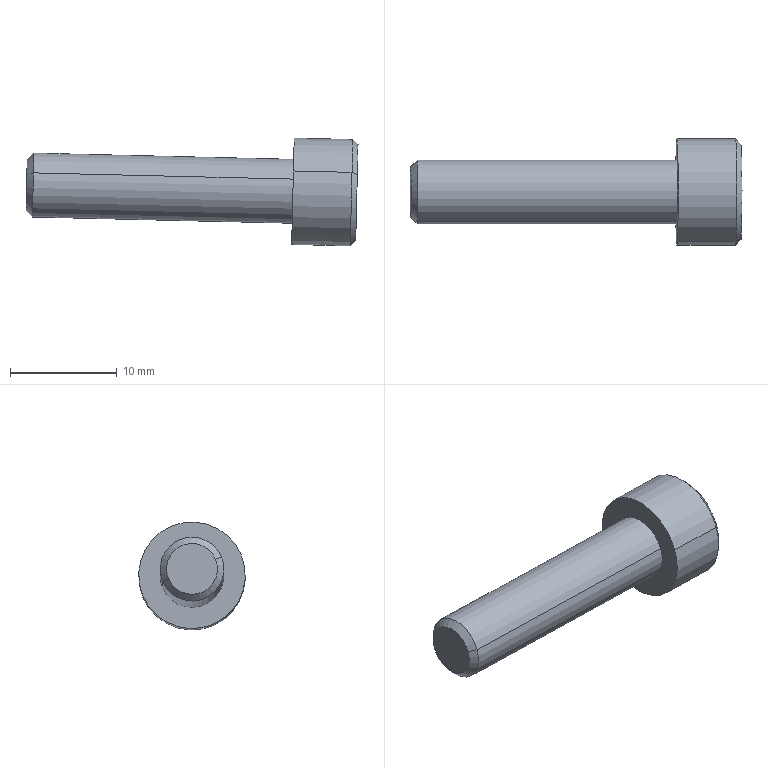Component | SolidWorks | 2012MB0201-1_AUpperRackFrameModule-1_ADJ42-G408-D6.5Assembly-10_HexSocketHeadCapScrewM6-25FerricOxide-1 | 1 solid | 25 faces | box 31.16 x 10 x 10.13 mm | volume 1097 mm3 | plane 15 | cone 6 | cylinder 4 | commonest cylinder face diameters 6 x2 10 x2 | material SCM435
STEP:
#1=COLOUR_RGB('',0.7922,0.8196,0.9333);
#2=FILL_AREA_STYLE_COLOUR('',#1);
#3=FILL_AREA_STYLE('',(#2));
#4=SURFACE_STYLE_FILL_AREA(#3);
#5=SURFACE_SIDE_STYLE('',(#4));
#6=SURFACE_STYLE_USAGE(.BOTH.,#5);
#7=PRESENTATION_STYLE_ASSIGNMENT((#6));
#8=CARTESIAN_POINT('',(-69.831,40.79,-44.912));
#9=VERTEX_POINT('',#8);
#10=CARTESIAN_POINT('',(-69.829,40.616,-44.84));
#11=VERTEX_POINT('',#10);
#12=CARTESIAN_POINT('',(-69.83,40.703,-44.876));
#13=DIRECTION('',(-0.9997,-0.,0.02392));
#14=DIRECTION('',(0.009134,-0.9242,0.3817));
#15=AXIS2_PLACEMENT_3D('',#12,#13,#14);
#16=CIRCLE('',#15,0.0939);
#17=EDGE_CURVE('',#9,#11,#16,.T.);
#18=ORIENTED_EDGE('',*,*,#17,.F.);
#19=CARTESIAN_POINT('',(-69.807,40.812,-44.922));
#20=VERTEX_POINT('',#19);
#21=CARTESIAN_POINT('',(-69.831,40.79,-44.912));
#22=DIRECTION('',(0.7004,0.6535,-0.2868));
#23=VECTOR('',#22,39.37);
#24=LINE('',#21,#23);
#25=EDGE_CURVE('',#9,#20,#24,.T.);
#26=ORIENTED_EDGE('',*,*,#25,.T.);
#27=CARTESIAN_POINT('',(-69.805,40.594,-44.832));
#28=VERTEX_POINT('',#27);
#29=CARTESIAN_POINT('',(-69.806,40.703,-44.877));
#30=DIRECTION('',(0.9997,0.,-0.02392));
#31=DIRECTION('',(0.009134,-0.9242,0.3817));
#32=AXIS2_PLACEMENT_3D('',#29,#30,#31);
#33=CIRCLE('',#32,0.1181);
#34=EDGE_CURVE('',#28,#20,#33,.T.);
#35=ORIENTED_EDGE('',*,*,#34,.F.);
#36=CARTESIAN_POINT('',(-69.829,40.616,-44.84));
#37=DIRECTION('',(0.7134,-0.6535,0.253));
#38=VECTOR('',#37,39.37);
#39=LINE('',#36,#38);
#40=EDGE_CURVE('',#11,#28,#39,.T.);
#41=ORIENTED_EDGE('',*,*,#40,.F.);
#42=EDGE_LOOP('',(#18,#26,#35,#41));
#43=FACE_OUTER_BOUND('',#42,.T.);
#44=CARTESIAN_POINT('',(-69.83,40.703,-44.876));
#45=DIRECTION('',(0.9997,0.,-0.02392));
#46=DIRECTION('',(0.009134,-0.9242,0.3817));
#47=AXIS2_PLACEMENT_3D('',#44,#45,#46);
#48=CONICAL_SURFACE('',#47,0.0939,0.7854);
#49=ADVANCED_FACE('',(#43),#48,.T.);
#50=ORIENTED_EDGE('',*,*,#34,.T.);
#51=CARTESIAN_POINT('',(-68.847,40.812,-44.945));
#52=VERTEX_POINT('',#51);
#53=CARTESIAN_POINT('',(-72.783,40.812,-44.851));
#54=DIRECTION('',(0.9997,0.,-0.02392));
#55=VECTOR('',#54,39.37);
#56=LINE('',#53,#55);
#57=EDGE_CURVE('',#20,#52,#56,.T.);
#58=ORIENTED_EDGE('',*,*,#57,.T.);
#59=CARTESIAN_POINT('',(-68.845,40.594,-44.855));
#60=VERTEX_POINT('',#59);
#61=CARTESIAN_POINT('',(-68.846,40.703,-44.9));
#62=DIRECTION('',(-0.9997,-0.,0.02392));
#63=DIRECTION('',(0.009134,-0.9242,0.3817));
#64=AXIS2_PLACEMENT_3D('',#61,#62,#63);
#65=CIRCLE('',#64,0.1181);
#66=EDGE_CURVE('',#52,#60,#65,.T.);
#67=ORIENTED_EDGE('',*,*,#66,.T.);
#68=CARTESIAN_POINT('',(-72.781,40.594,-44.76));
#69=DIRECTION('',(0.9997,0.,-0.02392));
#70=VECTOR('',#69,39.37);
#71=LINE('',#68,#70);
#72=EDGE_CURVE('',#28,#60,#71,.T.);
#73=ORIENTED_EDGE('',*,*,#72,.F.);
#74=EDGE_LOOP('',(#50,#58,#67,#73));
#75=FACE_OUTER_BOUND('',#74,.T.);
#76=CARTESIAN_POINT('',(-72.782,40.703,-44.806));
#77=DIRECTION('',(0.9997,0.,-0.02392));
#78=DIRECTION('',(0.009134,-0.9242,0.3817));
#79=AXIS2_PLACEMENT_3D('',#76,#77,#78);
#80=CYLINDRICAL_SURFACE('',#79,0.1181);
#81=ADVANCED_FACE('',(#75),#80,.T.);
#82=CARTESIAN_POINT('',(-68.844,40.521,-44.825));
#83=VERTEX_POINT('',#82);
#84=CARTESIAN_POINT('',(-68.848,40.885,-44.975));
#85=VERTEX_POINT('',#84);
#86=CARTESIAN_POINT('',(-68.846,40.703,-44.9));
#87=DIRECTION('',(0.9997,0.,-0.02392));
#88=DIRECTION('',(0.009134,-0.9242,0.3817));
#89=AXIS2_PLACEMENT_3D('',#86,#87,#88);
#90=CIRCLE('',#89,0.1969);
#91=EDGE_CURVE('',#83,#85,#90,.T.);
#92=ORIENTED_EDGE('',*,*,#91,.T.);
#93=CARTESIAN_POINT('',(-68.631,40.885,-44.98));
#94=VERTEX_POINT('',#93);
#95=CARTESIAN_POINT('',(-68.848,40.885,-44.975));
#96=DIRECTION('',(0.9997,0.,-0.02392));
#97=VECTOR('',#96,39.37);
#98=LINE('',#95,#97);
#99=EDGE_CURVE('',#85,#94,#98,.T.);
#100=ORIENTED_EDGE('',*,*,#99,.T.);
#101=CARTESIAN_POINT('',(-68.628,40.521,-44.83));
#102=VERTEX_POINT('',#101);
#103=CARTESIAN_POINT('',(-68.629,40.703,-44.905));
#104=DIRECTION('',(-0.9997,-0.,0.02392));
#105=DIRECTION('',(0.009134,-0.9242,0.3817));
#106=AXIS2_PLACEMENT_3D('',#103,#104,#105);
#107=CIRCLE('',#106,0.1969);
#108=EDGE_CURVE('',#94,#102,#107,.T.);
#109=ORIENTED_EDGE('',*,*,#108,.T.);
#110=CARTESIAN_POINT('',(-68.844,40.521,-44.825));
#111=DIRECTION('',(0.9997,0.,-0.02392));
#112=VECTOR('',#111,39.37);
#113=LINE('',#110,#112);
#114=EDGE_CURVE('',#83,#102,#113,.T.);
#115=ORIENTED_EDGE('',*,*,#114,.F.);
#116=EDGE_LOOP('',(#92,#100,#109,#115));
#117=FACE_OUTER_BOUND('',#116,.T.);
#118=CARTESIAN_POINT('',(-68.846,40.703,-44.9));
#119=DIRECTION('',(0.9997,0.,-0.02392));
#120=DIRECTION('',(0.009134,-0.9242,0.3817));
#121=AXIS2_PLACEMENT_3D('',#118,#119,#120);
#122=CYLINDRICAL_SURFACE('',#121,0.1969);
#123=ADVANCED_FACE('',(#117),#122,.T.);
#124=CARTESIAN_POINT('',(-68.611,40.867,-44.973));
#125=VERTEX_POINT('',#124);
#126=CARTESIAN_POINT('',(-68.608,40.539,-44.838));
#127=VERTEX_POINT('',#126);
#128=CARTESIAN_POINT('',(-68.61,40.703,-44.905));
#129=DIRECTION('',(-0.9997,-0.,0.02392));
#130=DIRECTION('',(-0.009134,0.9242,-0.3817));
#131=AXIS2_PLACEMENT_3D('',#128,#129,#130);
#132=CIRCLE('',#131,0.1772);
#133=EDGE_CURVE('',#125,#127,#132,.T.);
#134=ORIENTED_EDGE('',*,*,#133,.T.);
#135=CARTESIAN_POINT('',(-68.628,40.521,-44.83));
#136=DIRECTION('',(-0.7004,-0.6535,0.2868));
#137=VECTOR('',#136,39.37);
#138=LINE('',#135,#137);
#139=EDGE_CURVE('',#127,#102,#138,.T.);
#140=ORIENTED_EDGE('',*,*,#139,.T.);
#141=ORIENTED_EDGE('',*,*,#108,.F.);
#142=CARTESIAN_POINT('',(-68.631,40.885,-44.98));
#143=DIRECTION('',(-0.7134,0.6535,-0.253));
#144=VECTOR('',#143,39.37);
#145=LINE('',#142,#144);
#146=EDGE_CURVE('',#125,#94,#145,.T.);
#147=ORIENTED_EDGE('',*,*,#146,.F.);
#148=EDGE_LOOP('',(#134,#140,#141,#147));
#149=FACE_OUTER_BOUND('',#148,.T.);
#150=CARTESIAN_POINT('',(-68.629,40.703,-44.905));
#151=DIRECTION('',(-0.9997,-0.,0.02392));
#152=DIRECTION('',(-0.009134,0.9242,-0.3817));
#153=AXIS2_PLACEMENT_3D('',#150,#151,#152);
#154=CONICAL_SURFACE('',#153,0.1969,0.7854);
#155=ADVANCED_FACE('',(#149),#154,.T.);
#156=CARTESIAN_POINT('',(-68.785,40.703,-44.901));
#157=VERTEX_POINT('',#156);
#158=CARTESIAN_POINT('',(-68.727,40.612,-44.865));
#159=VERTEX_POINT('',#158);
#160=CARTESIAN_POINT('',(-68.727,40.612,-44.865));
#161=DIRECTION('',(0.5078,-0.8004,0.3186));
#162=VECTOR('',#161,39.37);
#163=LINE('',#160,#162);
#164=EDGE_CURVE('',#157,#159,#163,.T.);
#165=ORIENTED_EDGE('',*,*,#164,.F.);
#166=CARTESIAN_POINT('',(-68.729,40.794,-44.94));
#167=VERTEX_POINT('',#166);
#168=CARTESIAN_POINT('',(-68.729,40.794,-44.94));
#169=DIRECTION('',(0.4919,0.8004,-0.3426));
#170=VECTOR('',#169,39.37);
#171=LINE('',#168,#170);
#172=EDGE_CURVE('',#157,#167,#171,.T.);
#173=ORIENTED_EDGE('',*,*,#172,.T.);
#174=CARTESIAN_POINT('',(-68.726,40.781,-44.843));
#175=VERTEX_POINT('',#174);
#176=CARTESIAN_POINT('',(-68.728,40.703,-44.903));
#177=DIRECTION('',(-0.9997,-0.,0.02392));
#178=DIRECTION('',(0.009134,-0.9242,0.3817));
#179=AXIS2_PLACEMENT_3D('',#176,#177,#178);
#180=CIRCLE('',#179,0.09843);
#181=EDGE_CURVE('',#175,#167,#180,.T.);
#182=ORIENTED_EDGE('',*,*,#181,.F.);
#183=CARTESIAN_POINT('',(-68.725,40.69,-44.805));
#184=VERTEX_POINT('',#183);
#185=CARTESIAN_POINT('',(-68.728,40.703,-44.903));
#186=DIRECTION('',(-0.9997,-0.,0.02392));
#187=DIRECTION('',(0.009134,-0.9242,0.3817));
#188=AXIS2_PLACEMENT_3D('',#185,#186,#187);
#189=CIRCLE('',#188,0.09843);
#190=EDGE_CURVE('',#184,#175,#189,.T.);
#191=ORIENTED_EDGE('',*,*,#190,.F.);
#192=CARTESIAN_POINT('',(-68.728,40.703,-44.903));
#193=DIRECTION('',(-0.9997,-0.,0.02392));
#194=DIRECTION('',(0.009134,-0.9242,0.3817));
#195=AXIS2_PLACEMENT_3D('',#192,#193,#194);
#196=CIRCLE('',#195,0.09843);
#197=EDGE_CURVE('',#159,#184,#196,.T.);
#198=ORIENTED_EDGE('',*,*,#197,.F.);
#199=EDGE_LOOP('',(#165,#173,#182,#191,#198));
#200=FACE_OUTER_BOUND('',#199,.T.);
#201=CARTESIAN_POINT('',(-68.728,40.703,-44.903));
#202=DIRECTION('',(0.9997,0.,-0.02392));
#203=DIRECTION('',(0.009134,-0.9242,0.3817));
#204=AXIS2_PLACEMENT_3D('',#201,#202,#203);
#205=CONICAL_SURFACE('',#204,0.09843,1.047);
#206=ADVANCED_FACE('',(#200),#205,.F.);
#207=ORIENTED_EDGE('',*,*,#57,.F.);
#208=CARTESIAN_POINT('',(-69.806,40.703,-44.877));
#209=DIRECTION('',(0.9997,0.,-0.02392));
#210=DIRECTION('',(0.009134,-0.9242,0.3817));
#211=AXIS2_PLACEMENT_3D('',#208,#209,#210);
#212=CIRCLE('',#211,0.1181);
#213=EDGE_CURVE('',#20,#28,#212,.T.);
#214=ORIENTED_EDGE('',*,*,#213,.T.);
#215=ORIENTED_EDGE('',*,*,#72,.T.);
#216=CARTESIAN_POINT('',(-68.846,40.703,-44.9));
#217=DIRECTION('',(-0.9997,-0.,0.02392));
#218=DIRECTION('',(0.009134,-0.9242,0.3817));
#219=AXIS2_PLACEMENT_3D('',#216,#217,#218);
#220=CIRCLE('',#219,0.1181);
#221=EDGE_CURVE('',#60,#52,#220,.T.);
#222=ORIENTED_EDGE('',*,*,#221,.T.);
#223=EDGE_LOOP('',(#207,#214,#215,#222));
#224=FACE_OUTER_BOUND('',#223,.T.);
#225=CARTESIAN_POINT('',(-72.782,40.703,-44.806));
#226=DIRECTION('',(0.9997,0.,-0.02392));
#227=DIRECTION('',(0.009134,-0.9242,0.3817));
#228=AXIS2_PLACEMENT_3D('',#225,#226,#227);
#229=CYLINDRICAL_SURFACE('',#228,0.1181);
#230=ADVANCED_FACE('',(#224),#229,.T.);
#231=ORIENTED_EDGE('',*,*,#91,.F.);
#232=CARTESIAN_POINT('',(-68.846,40.703,-44.9));
#233=DIRECTION('',(0.9997,0.,-0.02392));
#234=DIRECTION('',(0.009134,-0.9242,0.3817));
#235=AXIS2_PLACEMENT_3D('',#232,#233,#234);
#236=CIRCLE('',#235,0.1969);
#237=EDGE_CURVE('',#85,#83,#236,.T.);
#238=ORIENTED_EDGE('',*,*,#237,.F.);
#239=EDGE_LOOP('',(#231,#238));
#240=FACE_OUTER_BOUND('',#239,.T.);
#241=ORIENTED_EDGE('',*,*,#221,.F.);
#242=ORIENTED_EDGE('',*,*,#66,.F.);
#243=EDGE_LOOP('',(#241,#242));
#244=FACE_BOUND('',#243,.T.);
#245=CARTESIAN_POINT('',(-68.85,40.628,-45.082));
#246=DIRECTION('',(0.9997,0.,-0.02392));
#247=DIRECTION('',(0.009134,-0.9242,0.3817));
#248=AXIS2_PLACEMENT_3D('',#245,#246,#247);
#249=PLANE('',#248);
#250=ADVANCED_FACE('',(#240,#244),#249,.F.);
#251=ORIENTED_EDGE('',*,*,#99,.F.);
#252=ORIENTED_EDGE('',*,*,#237,.T.);
#253=ORIENTED_EDGE('',*,*,#114,.T.);
#254=CARTESIAN_POINT('',(-68.629,40.703,-44.905));
#255=DIRECTION('',(-0.9997,-0.,0.02392));
#256=DIRECTION('',(0.009134,-0.9242,0.3817));
#257=AXIS2_PLACEMENT_3D('',#254,#255,#256);
#258=CIRCLE('',#257,0.1969);
#259=EDGE_CURVE('',#102,#94,#258,.T.);
#260=ORIENTED_EDGE('',*,*,#259,.T.);
#261=EDGE_LOOP('',(#251,#252,#253,#260));
#262=FACE_OUTER_BOUND('',#261,.T.);
#263=CARTESIAN_POINT('',(-68.846,40.703,-44.9));
#264=DIRECTION('',(0.9997,0.,-0.02392));
#265=DIRECTION('',(0.009134,-0.9242,0.3817));
#266=AXIS2_PLACEMENT_3D('',#263,#264,#265);
#267=CYLINDRICAL_SURFACE('',#266,0.1969);
#268=ADVANCED_FACE('',(#262),#267,.T.);
#269=ORIENTED_EDGE('',*,*,#139,.F.);
#270=CARTESIAN_POINT('',(-68.61,40.703,-44.905));
#271=DIRECTION('',(-0.9997,-0.,0.02392));
#272=DIRECTION('',(-0.009134,0.9242,-0.3817));
#273=AXIS2_PLACEMENT_3D('',#270,#271,#272);
#274=CIRCLE('',#273,0.1772);
#275=EDGE_CURVE('',#127,#125,#274,.T.);
#276=ORIENTED_EDGE('',*,*,#275,.T.);
#277=ORIENTED_EDGE('',*,*,#146,.T.);
#278=ORIENTED_EDGE('',*,*,#259,.F.);
#279=EDGE_LOOP('',(#269,#276,#277,#278));
#280=FACE_OUTER_BOUND('',#279,.T.);
#281=CARTESIAN_POINT('',(-68.629,40.703,-44.905));
#282=DIRECTION('',(-0.9997,-0.,0.02392));
#283=DIRECTION('',(-0.009134,0.9242,-0.3817));
#284=AXIS2_PLACEMENT_3D('',#281,#282,#283);
#285=CONICAL_SURFACE('',#284,0.1969,0.7854);
#286=ADVANCED_FACE('',(#280),#285,.T.);
#287=CARTESIAN_POINT('',(-68.609,40.815,-44.89));
#288=VERTEX_POINT('',#287);
#289=CARTESIAN_POINT('',(-68.607,40.746,-44.8));
#290=VERTEX_POINT('',#289);
#291=CARTESIAN_POINT('',(-68.609,40.815,-44.89));
#292=DIRECTION('',(0.01896,-0.6095,0.7926));
#293=VECTOR('',#292,39.37);
#294=LINE('',#291,#293);
#295=EDGE_CURVE('',#288,#290,#294,.T.);
#296=ORIENTED_EDGE('',*,*,#295,.F.);
#297=CARTESIAN_POINT('',(-68.612,40.772,-44.995));
#298=VERTEX_POINT('',#297);
#299=CARTESIAN_POINT('',(-68.611,40.794,-44.943));
#300=DIRECTION('',(0.02211,0.3818,0.924));
#301=VECTOR('',#300,39.37);
#302=LINE('',#299,#301);
#303=EDGE_CURVE('',#298,#288,#302,.T.);
#304=ORIENTED_EDGE('',*,*,#303,.F.);
#305=CARTESIAN_POINT('',(-68.612,40.659,-45.01));
#306=VERTEX_POINT('',#305);
#307=CARTESIAN_POINT('',(-68.612,40.659,-45.01));
#308=DIRECTION('',(0.003144,0.9913,0.1314));
#309=VECTOR('',#308,39.37);
#310=LINE('',#307,#309);
#311=EDGE_CURVE('',#306,#298,#310,.T.);
#312=ORIENTED_EDGE('',*,*,#311,.F.);
#313=CARTESIAN_POINT('',(-68.61,40.59,-44.92));
#314=VERTEX_POINT('',#313);
#315=CARTESIAN_POINT('',(-68.61,40.59,-44.92));
#316=DIRECTION('',(-0.01896,0.6095,-0.7926));
#317=VECTOR('',#316,39.37);
#318=LINE('',#315,#317);
#319=EDGE_CURVE('',#314,#306,#318,.T.);
#320=ORIENTED_EDGE('',*,*,#319,.F.);
#321=CARTESIAN_POINT('',(-68.608,40.634,-44.815));
#322=VERTEX_POINT('',#321);
#323=CARTESIAN_POINT('',(-68.609,40.612,-44.868));
#324=DIRECTION('',(-0.02211,-0.3818,-0.924));
#325=VECTOR('',#324,39.37);
#326=LINE('',#323,#325);
#327=EDGE_CURVE('',#322,#314,#326,.T.);
#328=ORIENTED_EDGE('',*,*,#327,.F.);
#329=CARTESIAN_POINT('',(-68.607,40.746,-44.8));
#330=DIRECTION('',(-0.003144,-0.9913,-0.1314));
#331=VECTOR('',#330,39.37);
#332=LINE('',#329,#331);
#333=EDGE_CURVE('',#290,#322,#332,.T.);
#334=ORIENTED_EDGE('',*,*,#333,.F.);
#335=EDGE_LOOP('',(#296,#304,#312,#320,#328,#334));
#336=FACE_BOUND('',#335,.T.);
#337=ORIENTED_EDGE('',*,*,#133,.F.);
#338=ORIENTED_EDGE('',*,*,#275,.F.);
#339=EDGE_LOOP('',(#337,#338));
#340=FACE_OUTER_BOUND('',#339,.T.);
#341=CARTESIAN_POINT('',(-68.61,40.703,-44.905));
#342=DIRECTION('',(-0.9997,-0.,0.02392));
#343=DIRECTION('',(-0.009134,0.9242,-0.3817));
#344=AXIS2_PLACEMENT_3D('',#341,#342,#343);
#345=PLANE('',#344);
#346=ADVANCED_FACE('',(#336,#340),#345,.F.);
#347=CARTESIAN_POINT('',(-68.726,40.634,-44.812));
#348=VERTEX_POINT('',#347);
#349=CARTESIAN_POINT('',(-68.726,40.634,-44.812));
#350=DIRECTION('',(0.9997,0.,-0.02392));
#351=VECTOR('',#350,39.37);
#352=LINE('',#349,#351);
#353=EDGE_CURVE('',#348,#322,#352,.T.);
#354=ORIENTED_EDGE('',*,*,#353,.F.);
#355=CARTESIAN_POINT('',(-68.725,40.69,-44.805));
#356=DIRECTION('',(-0.003144,-0.9913,-0.1314));
#357=VECTOR('',#356,39.37);
#358=LINE('',#355,#357);
#359=EDGE_CURVE('',#184,#348,#358,.T.);
#360=ORIENTED_EDGE('',*,*,#359,.F.);
#361=CARTESIAN_POINT('',(-68.725,40.746,-44.798));
#362=VERTEX_POINT('',#361);
#363=CARTESIAN_POINT('',(-68.725,40.746,-44.798));
#364=DIRECTION('',(-0.003144,-0.9913,-0.1314));
#365=VECTOR('',#364,39.37);
#366=LINE('',#363,#365);
#367=EDGE_CURVE('',#362,#184,#366,.T.);
#368=ORIENTED_EDGE('',*,*,#367,.F.);
#369=CARTESIAN_POINT('',(-68.725,40.746,-44.798));
#370=DIRECTION('',(-0.9997,-0.,0.02392));
#371=VECTOR('',#370,39.37);
#372=LINE('',#369,#371);
#373=EDGE_CURVE('',#290,#362,#372,.T.);
#374=ORIENTED_EDGE('',*,*,#373,.F.);
#375=ORIENTED_EDGE('',*,*,#333,.T.);
#376=EDGE_LOOP('',(#354,#360,#368,#374,#375));
#377=FACE_OUTER_BOUND('',#376,.T.);
#378=CARTESIAN_POINT('',(-68.725,40.746,-44.798));
#379=DIRECTION('',(0.02371,-0.1314,0.991));
#380=DIRECTION('',(-0.003144,-0.9913,-0.1314));
#381=AXIS2_PLACEMENT_3D('',#378,#379,#380);
#382=PLANE('',#381);
#383=ADVANCED_FACE('',(#377),#382,.F.);
#384=ORIENTED_EDGE('',*,*,#373,.T.);
#385=CARTESIAN_POINT('',(-68.726,40.781,-44.843));
#386=DIRECTION('',(0.01896,-0.6095,0.7926));
#387=VECTOR('',#386,39.37);
#388=LINE('',#385,#387);
#389=EDGE_CURVE('',#175,#362,#388,.T.);
#390=ORIENTED_EDGE('',*,*,#389,.F.);
#391=CARTESIAN_POINT('',(-68.727,40.815,-44.888));
#392=VERTEX_POINT('',#391);
#393=CARTESIAN_POINT('',(-68.727,40.815,-44.888));
#394=DIRECTION('',(0.01896,-0.6095,0.7926));
#395=VECTOR('',#394,39.37);
#396=LINE('',#393,#395);
#397=EDGE_CURVE('',#392,#175,#396,.T.);
#398=ORIENTED_EDGE('',*,*,#397,.F.);
#399=CARTESIAN_POINT('',(-68.727,40.815,-44.888));
#400=DIRECTION('',(-0.9997,-0.,0.02392));
#401=VECTOR('',#400,39.37);
#402=LINE('',#399,#401);
#403=EDGE_CURVE('',#288,#392,#402,.T.);
#404=ORIENTED_EDGE('',*,*,#403,.F.);
#405=ORIENTED_EDGE('',*,*,#295,.T.);
#406=EDGE_LOOP('',(#384,#390,#398,#404,#405));
#407=FACE_OUTER_BOUND('',#406,.T.);
#408=CARTESIAN_POINT('',(-68.727,40.815,-44.888));
#409=DIRECTION('',(0.01458,0.7928,0.6093));
#410=DIRECTION('',(0.01896,-0.6095,0.7926));
#411=AXIS2_PLACEMENT_3D('',#408,#409,#410);
#412=PLANE('',#411);
#413=ADVANCED_FACE('',(#407),#412,.F.);
#414=ORIENTED_EDGE('',*,*,#403,.T.);
#415=CARTESIAN_POINT('',(-68.729,40.794,-44.94));
#416=DIRECTION('',(0.02211,0.3818,0.924));
#417=VECTOR('',#416,39.37);
#418=LINE('',#415,#417);
#419=EDGE_CURVE('',#167,#392,#418,.T.);
#420=ORIENTED_EDGE('',*,*,#419,.F.);
#421=CARTESIAN_POINT('',(-68.73,40.772,-44.993));
#422=VERTEX_POINT('',#421);
#423=CARTESIAN_POINT('',(-68.729,40.794,-44.94));
#424=DIRECTION('',(0.02211,0.3818,0.924));
#425=VECTOR('',#424,39.37);
#426=LINE('',#423,#425);
#427=EDGE_CURVE('',#422,#167,#426,.T.);
#428=ORIENTED_EDGE('',*,*,#427,.F.);
#429=CARTESIAN_POINT('',(-68.73,40.772,-44.993));
#430=DIRECTION('',(-0.9997,-0.,0.02392));
#431=VECTOR('',#430,39.37);
#432=LINE('',#429,#431);
#433=EDGE_CURVE('',#298,#422,#432,.T.);
#434=ORIENTED_EDGE('',*,*,#433,.F.);
#435=ORIENTED_EDGE('',*,*,#303,.T.);
#436=EDGE_LOOP('',(#414,#420,#428,#434,#435));
#437=FACE_OUTER_BOUND('',#436,.T.);
#438=CARTESIAN_POINT('',(-68.73,40.772,-44.993));
#439=DIRECTION('',(-0.009134,0.9242,-0.3817));
#440=DIRECTION('',(0.9997,0.,-0.02392));
#441=AXIS2_PLACEMENT_3D('',#438,#439,#440);
#442=PLANE('',#441);
#443=ADVANCED_FACE('',(#437),#442,.F.);
#444=ORIENTED_EDGE('',*,*,#433,.T.);
#445=CARTESIAN_POINT('',(-68.73,40.716,-45.));
#446=VERTEX_POINT('',#445);
#447=CARTESIAN_POINT('',(-68.73,40.716,-45.));
#448=DIRECTION('',(0.003144,0.9913,0.1314));
#449=VECTOR('',#448,39.37);
#450=LINE('',#447,#449);
#451=EDGE_CURVE('',#446,#422,#450,.T.);
#452=ORIENTED_EDGE('',*,*,#451,.F.);
#453=CARTESIAN_POINT('',(-68.73,40.659,-45.008));
#454=VERTEX_POINT('',#453);
#455=CARTESIAN_POINT('',(-68.73,40.659,-45.008));
#456=DIRECTION('',(0.003144,0.9913,0.1314));
#457=VECTOR('',#456,39.37);
#458=LINE('',#455,#457);
#459=EDGE_CURVE('',#454,#446,#458,.T.);
#460=ORIENTED_EDGE('',*,*,#459,.F.);
#461=CARTESIAN_POINT('',(-68.73,40.659,-45.008));
#462=DIRECTION('',(-0.9997,-0.,0.02392));
#463=VECTOR('',#462,39.37);
#464=LINE('',#461,#463);
#465=EDGE_CURVE('',#306,#454,#464,.T.);
#466=ORIENTED_EDGE('',*,*,#465,.F.);
#467=ORIENTED_EDGE('',*,*,#311,.T.);
#468=EDGE_LOOP('',(#444,#452,#460,#466,#467));
#469=FACE_OUTER_BOUND('',#468,.T.);
#470=CARTESIAN_POINT('',(-68.73,40.659,-45.008));
#471=DIRECTION('',(-0.02371,0.1314,-0.991));
#472=DIRECTION('',(0.003144,0.9913,0.1314));
#473=AXIS2_PLACEMENT_3D('',#470,#471,#472);
#474=PLANE('',#473);
#475=ADVANCED_FACE('',(#469),#474,.F.);
#476=ORIENTED_EDGE('',*,*,#465,.T.);
#477=CARTESIAN_POINT('',(-68.729,40.625,-44.963));
#478=VERTEX_POINT('',#477);
#479=CARTESIAN_POINT('',(-68.729,40.625,-44.963));
#480=DIRECTION('',(-0.01896,0.6095,-0.7926));
#481=VECTOR('',#480,39.37);
#482=LINE('',#479,#481);
#483=EDGE_CURVE('',#478,#454,#482,.T.);
#484=ORIENTED_EDGE('',*,*,#483,.F.);
#485=CARTESIAN_POINT('',(-68.728,40.59,-44.918));
#486=VERTEX_POINT('',#485);
#487=CARTESIAN_POINT('',(-68.728,40.59,-44.918));
#488=DIRECTION('',(-0.01896,0.6095,-0.7926));
#489=VECTOR('',#488,39.37);
#490=LINE('',#487,#489);
#491=EDGE_CURVE('',#486,#478,#490,.T.);
#492=ORIENTED_EDGE('',*,*,#491,.F.);
#493=CARTESIAN_POINT('',(-68.728,40.59,-44.918));
#494=DIRECTION('',(-0.9997,-0.,0.02392));
#495=VECTOR('',#494,39.37);
#496=LINE('',#493,#495);
#497=EDGE_CURVE('',#314,#486,#496,.T.);
#498=ORIENTED_EDGE('',*,*,#497,.F.);
#499=ORIENTED_EDGE('',*,*,#319,.T.);
#500=EDGE_LOOP('',(#476,#484,#492,#498,#499));
#501=FACE_OUTER_BOUND('',#500,.T.);
#502=CARTESIAN_POINT('',(-68.728,40.59,-44.918));
#503=DIRECTION('',(-0.01458,-0.7928,-0.6093));
#504=DIRECTION('',(-0.01896,0.6095,-0.7926));
#505=AXIS2_PLACEMENT_3D('',#502,#503,#504);
#506=PLANE('',#505);
#507=ADVANCED_FACE('',(#501),#506,.F.);
#508=ORIENTED_EDGE('',*,*,#497,.T.);
#509=CARTESIAN_POINT('',(-68.726,40.634,-44.812));
#510=DIRECTION('',(-0.02211,-0.3818,-0.924));
#511=VECTOR('',#510,39.37);
#512=LINE('',#509,#511);
#513=EDGE_CURVE('',#159,#486,#512,.T.);
#514=ORIENTED_EDGE('',*,*,#513,.F.);
#515=CARTESIAN_POINT('',(-68.727,40.612,-44.865));
#516=DIRECTION('',(-0.02211,-0.3818,-0.924));
#517=VECTOR('',#516,39.37);
#518=LINE('',#515,#517);
#519=EDGE_CURVE('',#348,#159,#518,.T.);
#520=ORIENTED_EDGE('',*,*,#519,.F.);
#521=ORIENTED_EDGE('',*,*,#353,.T.);
#522=ORIENTED_EDGE('',*,*,#327,.T.);
#523=EDGE_LOOP('',(#508,#514,#520,#521,#522));
#524=FACE_OUTER_BOUND('',#523,.T.);
#525=CARTESIAN_POINT('',(-68.726,40.634,-44.812));
#526=DIRECTION('',(0.009134,-0.9242,0.3817));
#527=DIRECTION('',(-0.9997,-0.,0.02392));
#528=AXIS2_PLACEMENT_3D('',#525,#526,#527);
#529=PLANE('',#528);
#530=ADVANCED_FACE('',(#524),#529,.F.);
#531=CARTESIAN_POINT('',(-68.728,40.703,-44.903));
#532=DIRECTION('',(-0.9997,-0.,0.02392));
#533=DIRECTION('',(0.009134,-0.9242,0.3817));
#534=AXIS2_PLACEMENT_3D('',#531,#532,#533);
#535=CIRCLE('',#534,0.09843);
#536=EDGE_CURVE('',#478,#159,#535,.T.);
#537=ORIENTED_EDGE('',*,*,#536,.T.);
#538=ORIENTED_EDGE('',*,*,#513,.T.);
#539=ORIENTED_EDGE('',*,*,#491,.T.);
#540=EDGE_LOOP('',(#537,#538,#539));
#541=FACE_OUTER_BOUND('',#540,.T.);
#542=CARTESIAN_POINT('',(-68.728,40.703,-44.903));
#543=DIRECTION('',(0.9997,0.,-0.02392));
#544=DIRECTION('',(0.009134,-0.9242,0.3817));
#545=AXIS2_PLACEMENT_3D('',#542,#543,#544);
#546=PLANE('',#545);
#547=ADVANCED_FACE('',(#541),#546,.T.);
#548=ORIENTED_EDGE('',*,*,#172,.F.);
#549=ORIENTED_EDGE('',*,*,#164,.T.);
#550=ORIENTED_EDGE('',*,*,#536,.F.);
#551=CARTESIAN_POINT('',(-68.728,40.703,-44.903));
#552=DIRECTION('',(-0.9997,-0.,0.02392));
#553=DIRECTION('',(0.009134,-0.9242,0.3817));
#554=AXIS2_PLACEMENT_3D('',#551,#552,#553);
#555=CIRCLE('',#554,0.09843);
#556=EDGE_CURVE('',#446,#478,#555,.T.);
#557=ORIENTED_EDGE('',*,*,#556,.F.);
#558=CARTESIAN_POINT('',(-68.728,40.703,-44.903));
#559=DIRECTION('',(-0.9997,-0.,0.02392));
#560=DIRECTION('',(0.009134,-0.9242,0.3817));
#561=AXIS2_PLACEMENT_3D('',#558,#559,#560);
#562=CIRCLE('',#561,0.09843);
#563=EDGE_CURVE('',#167,#446,#562,.T.);
#564=ORIENTED_EDGE('',*,*,#563,.F.);
#565=EDGE_LOOP('',(#548,#549,#550,#557,#564));
#566=FACE_OUTER_BOUND('',#565,.T.);
#567=CARTESIAN_POINT('',(-68.728,40.703,-44.903));
#568=DIRECTION('',(0.9997,0.,-0.02392));
#569=DIRECTION('',(0.009134,-0.9242,0.3817));
#570=AXIS2_PLACEMENT_3D('',#567,#568,#569);
#571=CONICAL_SURFACE('',#570,0.09843,1.047);
#572=ADVANCED_FACE('',(#566),#571,.F.);
#573=ORIENTED_EDGE('',*,*,#556,.T.);
#574=ORIENTED_EDGE('',*,*,#483,.T.);
#575=ORIENTED_EDGE('',*,*,#459,.T.);
#576=EDGE_LOOP('',(#573,#574,#575));
#577=FACE_OUTER_BOUND('',#576,.T.);
#578=CARTESIAN_POINT('',(-68.728,40.703,-44.903));
#579=DIRECTION('',(0.9997,0.,-0.02392));
#580=DIRECTION('',(0.009134,-0.9242,0.3817));
#581=AXIS2_PLACEMENT_3D('',#578,#579,#580);
#582=PLANE('',#581);
#583=ADVANCED_FACE('',(#577),#582,.T.);
#584=ORIENTED_EDGE('',*,*,#563,.T.);
#585=ORIENTED_EDGE('',*,*,#451,.T.);
#586=ORIENTED_EDGE('',*,*,#427,.T.);
#587=EDGE_LOOP('',(#584,#585,#586));
#588=FACE_OUTER_BOUND('',#587,.T.);
#589=CARTESIAN_POINT('',(-68.728,40.703,-44.903));
#590=DIRECTION('',(0.9997,0.,-0.02392));
#591=DIRECTION('',(0.009134,-0.9242,0.3817));
#592=AXIS2_PLACEMENT_3D('',#589,#590,#591);
#593=PLANE('',#592);
#594=ADVANCED_FACE('',(#588),#593,.T.);
#595=ORIENTED_EDGE('',*,*,#181,.T.);
#596=ORIENTED_EDGE('',*,*,#419,.T.);
#597=ORIENTED_EDGE('',*,*,#397,.T.);
#598=EDGE_LOOP('',(#595,#596,#597));
#599=FACE_OUTER_BOUND('',#598,.T.);
#600=CARTESIAN_POINT('',(-68.728,40.703,-44.903));
#601=DIRECTION('',(0.9997,0.,-0.02392));
#602=DIRECTION('',(0.009134,-0.9242,0.3817));
#603=AXIS2_PLACEMENT_3D('',#600,#601,#602);
#604=PLANE('',#603);
#605=ADVANCED_FACE('',(#599),#604,.T.);
#606=ORIENTED_EDGE('',*,*,#190,.T.);
#607=ORIENTED_EDGE('',*,*,#389,.T.);
#608=ORIENTED_EDGE('',*,*,#367,.T.);
#609=EDGE_LOOP('',(#606,#607,#608));
#610=FACE_OUTER_BOUND('',#609,.T.);
#611=CARTESIAN_POINT('',(-68.728,40.703,-44.903));
#612=DIRECTION('',(0.9997,0.,-0.02392));
#613=DIRECTION('',(0.009134,-0.9242,0.3817));
#614=AXIS2_PLACEMENT_3D('',#611,#612,#613);
#615=PLANE('',#614);
#616=ADVANCED_FACE('',(#610),#615,.T.);
#617=ORIENTED_EDGE('',*,*,#197,.T.);
#618=ORIENTED_EDGE('',*,*,#359,.T.);
#619=ORIENTED_EDGE('',*,*,#519,.T.);
#620=EDGE_LOOP('',(#617,#618,#619));
#621=FACE_OUTER_BOUND('',#620,.T.);
#622=CARTESIAN_POINT('',(-68.728,40.703,-44.903));
#623=DIRECTION('',(0.9997,0.,-0.02392));
#624=DIRECTION('',(0.009134,-0.9242,0.3817));
#625=AXIS2_PLACEMENT_3D('',#622,#623,#624);
#626=PLANE('',#625);
#627=ADVANCED_FACE('',(#621),#626,.T.);
#628=CARTESIAN_POINT('',(-69.83,40.703,-44.876));
#629=DIRECTION('',(-0.9997,-0.,0.02392));
#630=DIRECTION('',(0.009134,-0.9242,0.3817));
#631=AXIS2_PLACEMENT_3D('',#628,#629,#630);
#632=CIRCLE('',#631,0.0939);
#633=EDGE_CURVE('',#11,#9,#632,.T.);
#634=ORIENTED_EDGE('',*,*,#633,.T.);
#635=ORIENTED_EDGE('',*,*,#17,.T.);
#636=EDGE_LOOP('',(#634,#635));
#637=FACE_OUTER_BOUND('',#636,.T.);
#638=CARTESIAN_POINT('',(-69.841,40.725,-45.338));
#639=DIRECTION('',(0.9997,0.,-0.02392));
#640=DIRECTION('',(0.009134,-0.9242,0.3817));
#641=AXIS2_PLACEMENT_3D('',#638,#639,#640);
#642=PLANE('',#641);
#643=ADVANCED_FACE('',(#637),#642,.F.);
#644=ORIENTED_EDGE('',*,*,#25,.F.);
#645=ORIENTED_EDGE('',*,*,#633,.F.);
#646=ORIENTED_EDGE('',*,*,#40,.T.);
#647=ORIENTED_EDGE('',*,*,#213,.F.);
#648=EDGE_LOOP('',(#644,#645,#646,#647));
#649=FACE_OUTER_BOUND('',#648,.T.);
#650=CARTESIAN_POINT('',(-69.83,40.703,-44.876));
#651=DIRECTION('',(0.9997,0.,-0.02392));
#652=DIRECTION('',(0.009134,-0.9242,0.3817));
#653=AXIS2_PLACEMENT_3D('',#650,#651,#652);
#654=CONICAL_SURFACE('',#653,0.0939,0.7854);
#655=ADVANCED_FACE('',(#649),#654,.T.);
#656=CLOSED_SHELL('',(#49,#81,#123,#155,#206,#230,#250,#268,#286,#346,#383,#413,#443,#475,#507,#530,#547,#572,#583,#594,#605,#616,#627,#643,#655));
#657=MANIFOLD_SOLID_BREP('',#656);
#658=STYLED_ITEM('',(#7),#657);
#659=PRESENTATION_LAYER_ASSIGNMENT('','',(#658));
#660=CARTESIAN_POINT('',(0.,0.,0.));
#661=DIRECTION('',(0.,0.,1.));
#662=DIRECTION('',(1.,0.,0.));
#663=AXIS2_PLACEMENT_3D('',#660,#661,#662);
#664=(LENGTH_UNIT()NAMED_UNIT(*)SI_UNIT($,.METRE.));
#665=LENGTH_MEASURE_WITH_UNIT(LENGTH_MEASURE(0.0254),#664);
#666=DIMENSIONAL_EXPONENTS(1.,0.,0.,0.,0.,0.,0.);
#667=(CONVERSION_BASED_UNIT('',#665)LENGTH_UNIT()NAMED_UNIT(#666));
#668=UNCERTAINTY_MEASURE_WITH_UNIT(LENGTH_MEASURE(0.00001),#667,'','');
#669=(NAMED_UNIT(*)PLANE_ANGLE_UNIT()SI_UNIT($,.RADIAN.));
#670=(NAMED_UNIT(*)SI_UNIT($,.STERADIAN.)SOLID_ANGLE_UNIT());
#671=(GEOMETRIC_REPRESENTATION_CONTEXT(3)GLOBAL_UNCERTAINTY_ASSIGNED_CONTEXT((#668))GLOBAL_UNIT_ASSIGNED_CONTEXT((#667,#669,#670))REPRESENTATION_CONTEXT('',''));
#672=ADVANCED_BREP_SHAPE_REPRESENTATION('',(#657,#663),#671);
#673=(LENGTH_UNIT()NAMED_UNIT(*)SI_UNIT($,.METRE.));
#674=LENGTH_MEASURE_WITH_UNIT(LENGTH_MEASURE(0.0254),#673);
#675=DIMENSIONAL_EXPONENTS(1.,0.,0.,0.,0.,0.,0.);
#676=(CONVERSION_BASED_UNIT('',#674)LENGTH_UNIT()NAMED_UNIT(#675));
#677=UNCERTAINTY_MEASURE_WITH_UNIT(LENGTH_MEASURE(0.00001),#676,'','');
#678=(NAMED_UNIT(*)PLANE_ANGLE_UNIT()SI_UNIT($,.RADIAN.));
#679=(NAMED_UNIT(*)SI_UNIT($,.STERADIAN.)SOLID_ANGLE_UNIT());
#680=(GEOMETRIC_REPRESENTATION_CONTEXT(3)GLOBAL_UNCERTAINTY_ASSIGNED_CONTEXT((#677))GLOBAL_UNIT_ASSIGNED_CONTEXT((#676,#678,#679))REPRESENTATION_CONTEXT('',''));
#681=MECHANICAL_DESIGN_GEOMETRIC_PRESENTATION_REPRESENTATION('',(#658),#680);